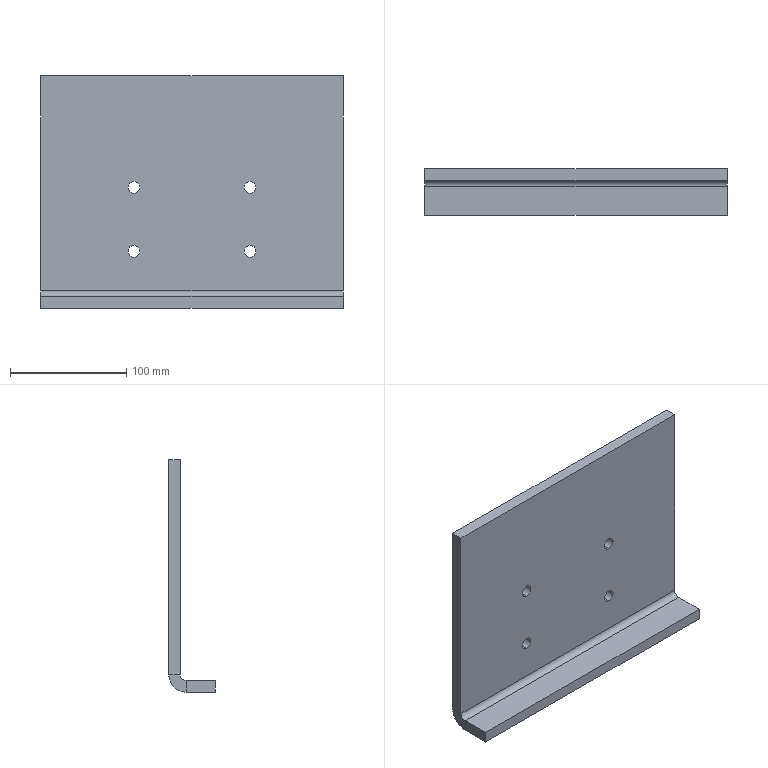Component | SolidWorks | THK-A1017LeftAndRightRectangularTubeConnectingPlate-1 | 1 solid | 22 faces | box 260 x 40 x 200 mm | volume 583572 mm3 | plane 12 | cylinder 10 | commonest cylinder face diameters 10.2 x8 30 x1 10 x1 | material Q235A
STEP:
#1=CARTESIAN_POINT('',(1.969,-2.953,-28.421));
#2=VERTEX_POINT('',#1);
#3=CARTESIAN_POINT('',(1.969,-2.953,-28.823));
#4=VERTEX_POINT('',#3);
#5=CARTESIAN_POINT('',(1.969,-2.953,-28.622));
#6=DIRECTION('',(0.,-1.,0.));
#7=DIRECTION('',(0.,0.,-1.));
#8=AXIS2_PLACEMENT_3D('',#5,#6,#7);
#9=CIRCLE('',#8,0.2008);
#10=EDGE_CURVE('',#2,#4,#9,.T.);
#11=ORIENTED_EDGE('',*,*,#10,.F.);
#12=CARTESIAN_POINT('',(1.969,-3.346,-28.421));
#13=VERTEX_POINT('',#12);
#14=CARTESIAN_POINT('',(1.969,-3.346,-28.421));
#15=DIRECTION('',(0.,-1.,0.));
#16=VECTOR('',#15,39.37);
#17=LINE('',#14,#16);
#18=EDGE_CURVE('',#2,#13,#17,.T.);
#19=ORIENTED_EDGE('',*,*,#18,.T.);
#20=CARTESIAN_POINT('',(1.969,-3.346,-28.823));
#21=VERTEX_POINT('',#20);
#22=CARTESIAN_POINT('',(1.969,-3.346,-28.622));
#23=DIRECTION('',(0.,-1.,0.));
#24=DIRECTION('',(0.,0.,-1.));
#25=AXIS2_PLACEMENT_3D('',#22,#23,#24);
#26=CIRCLE('',#25,0.2008);
#27=EDGE_CURVE('',#13,#21,#26,.T.);
#28=ORIENTED_EDGE('',*,*,#27,.T.);
#29=CARTESIAN_POINT('',(1.969,-3.346,-28.823));
#30=DIRECTION('',(0.,-1.,0.));
#31=VECTOR('',#30,39.37);
#32=LINE('',#29,#31);
#33=EDGE_CURVE('',#4,#21,#32,.T.);
#34=ORIENTED_EDGE('',*,*,#33,.F.);
#35=EDGE_LOOP('',(#11,#19,#28,#34));
#36=FACE_OUTER_BOUND('',#35,.T.);
#37=CARTESIAN_POINT('',(1.969,-3.346,-28.622));
#38=DIRECTION('',(0.,-1.,0.));
#39=DIRECTION('',(0.,0.,-1.));
#40=AXIS2_PLACEMENT_3D('',#37,#38,#39);
#41=CYLINDRICAL_SURFACE('',#40,0.2008);
#42=ADVANCED_FACE('',(#36),#41,.F.);
#43=CARTESIAN_POINT('',(1.969,-2.953,-26.256));
#44=VERTEX_POINT('',#43);
#45=CARTESIAN_POINT('',(1.969,-2.953,-26.657));
#46=VERTEX_POINT('',#45);
#47=CARTESIAN_POINT('',(1.969,-2.953,-26.457));
#48=DIRECTION('',(0.,-1.,0.));
#49=DIRECTION('',(0.,0.,-1.));
#50=AXIS2_PLACEMENT_3D('',#47,#48,#49);
#51=CIRCLE('',#50,0.2008);
#52=EDGE_CURVE('',#44,#46,#51,.T.);
#53=ORIENTED_EDGE('',*,*,#52,.F.);
#54=CARTESIAN_POINT('',(1.969,-3.346,-26.256));
#55=VERTEX_POINT('',#54);
#56=CARTESIAN_POINT('',(1.969,-3.346,-26.256));
#57=DIRECTION('',(0.,-1.,0.));
#58=VECTOR('',#57,39.37);
#59=LINE('',#56,#58);
#60=EDGE_CURVE('',#44,#55,#59,.T.);
#61=ORIENTED_EDGE('',*,*,#60,.T.);
#62=CARTESIAN_POINT('',(1.969,-3.346,-26.657));
#63=VERTEX_POINT('',#62);
#64=CARTESIAN_POINT('',(1.969,-3.346,-26.457));
#65=DIRECTION('',(0.,-1.,0.));
#66=DIRECTION('',(0.,0.,-1.));
#67=AXIS2_PLACEMENT_3D('',#64,#65,#66);
#68=CIRCLE('',#67,0.2008);
#69=EDGE_CURVE('',#55,#63,#68,.T.);
#70=ORIENTED_EDGE('',*,*,#69,.T.);
#71=CARTESIAN_POINT('',(1.969,-3.346,-26.657));
#72=DIRECTION('',(0.,-1.,0.));
#73=VECTOR('',#72,39.37);
#74=LINE('',#71,#73);
#75=EDGE_CURVE('',#46,#63,#74,.T.);
#76=ORIENTED_EDGE('',*,*,#75,.F.);
#77=EDGE_LOOP('',(#53,#61,#70,#76));
#78=FACE_OUTER_BOUND('',#77,.T.);
#79=CARTESIAN_POINT('',(1.969,-3.346,-26.457));
#80=DIRECTION('',(0.,-1.,0.));
#81=DIRECTION('',(0.,0.,-1.));
#82=AXIS2_PLACEMENT_3D('',#79,#80,#81);
#83=CYLINDRICAL_SURFACE('',#82,0.2008);
#84=ADVANCED_FACE('',(#78),#83,.F.);
#85=CARTESIAN_POINT('',(-1.969,-2.953,-26.256));
#86=VERTEX_POINT('',#85);
#87=CARTESIAN_POINT('',(-1.969,-2.953,-26.657));
#88=VERTEX_POINT('',#87);
#89=CARTESIAN_POINT('',(-1.969,-2.953,-26.457));
#90=DIRECTION('',(0.,-1.,0.));
#91=DIRECTION('',(0.,0.,-1.));
#92=AXIS2_PLACEMENT_3D('',#89,#90,#91);
#93=CIRCLE('',#92,0.2008);
#94=EDGE_CURVE('',#86,#88,#93,.T.);
#95=ORIENTED_EDGE('',*,*,#94,.F.);
#96=CARTESIAN_POINT('',(-1.969,-3.346,-26.256));
#97=VERTEX_POINT('',#96);
#98=CARTESIAN_POINT('',(-1.969,-3.346,-26.256));
#99=DIRECTION('',(0.,-1.,0.));
#100=VECTOR('',#99,39.37);
#101=LINE('',#98,#100);
#102=EDGE_CURVE('',#86,#97,#101,.T.);
#103=ORIENTED_EDGE('',*,*,#102,.T.);
#104=CARTESIAN_POINT('',(-1.969,-3.346,-26.657));
#105=VERTEX_POINT('',#104);
#106=CARTESIAN_POINT('',(-1.969,-3.346,-26.457));
#107=DIRECTION('',(0.,-1.,0.));
#108=DIRECTION('',(0.,0.,-1.));
#109=AXIS2_PLACEMENT_3D('',#106,#107,#108);
#110=CIRCLE('',#109,0.2008);
#111=EDGE_CURVE('',#97,#105,#110,.T.);
#112=ORIENTED_EDGE('',*,*,#111,.T.);
#113=CARTESIAN_POINT('',(-1.969,-3.346,-26.657));
#114=DIRECTION('',(0.,-1.,0.));
#115=VECTOR('',#114,39.37);
#116=LINE('',#113,#115);
#117=EDGE_CURVE('',#88,#105,#116,.T.);
#118=ORIENTED_EDGE('',*,*,#117,.F.);
#119=EDGE_LOOP('',(#95,#103,#112,#118));
#120=FACE_OUTER_BOUND('',#119,.T.);
#121=CARTESIAN_POINT('',(-1.969,-3.346,-26.457));
#122=DIRECTION('',(0.,-1.,0.));
#123=DIRECTION('',(0.,0.,-1.));
#124=AXIS2_PLACEMENT_3D('',#121,#122,#123);
#125=CYLINDRICAL_SURFACE('',#124,0.2008);
#126=ADVANCED_FACE('',(#120),#125,.F.);
#127=CARTESIAN_POINT('',(-1.969,-2.953,-28.421));
#128=VERTEX_POINT('',#127);
#129=CARTESIAN_POINT('',(-1.969,-2.953,-28.823));
#130=VERTEX_POINT('',#129);
#131=CARTESIAN_POINT('',(-1.969,-2.953,-28.622));
#132=DIRECTION('',(0.,-1.,0.));
#133=DIRECTION('',(0.,0.,-1.));
#134=AXIS2_PLACEMENT_3D('',#131,#132,#133);
#135=CIRCLE('',#134,0.2008);
#136=EDGE_CURVE('',#128,#130,#135,.T.);
#137=ORIENTED_EDGE('',*,*,#136,.F.);
#138=CARTESIAN_POINT('',(-1.969,-3.346,-28.421));
#139=VERTEX_POINT('',#138);
#140=CARTESIAN_POINT('',(-1.969,-3.346,-28.421));
#141=DIRECTION('',(0.,-1.,0.));
#142=VECTOR('',#141,39.37);
#143=LINE('',#140,#142);
#144=EDGE_CURVE('',#128,#139,#143,.T.);
#145=ORIENTED_EDGE('',*,*,#144,.T.);
#146=CARTESIAN_POINT('',(-1.969,-3.346,-28.823));
#147=VERTEX_POINT('',#146);
#148=CARTESIAN_POINT('',(-1.969,-3.346,-28.622));
#149=DIRECTION('',(0.,-1.,0.));
#150=DIRECTION('',(0.,0.,-1.));
#151=AXIS2_PLACEMENT_3D('',#148,#149,#150);
#152=CIRCLE('',#151,0.2008);
#153=EDGE_CURVE('',#139,#147,#152,.T.);
#154=ORIENTED_EDGE('',*,*,#153,.T.);
#155=CARTESIAN_POINT('',(-1.969,-3.346,-28.823));
#156=DIRECTION('',(0.,-1.,0.));
#157=VECTOR('',#156,39.37);
#158=LINE('',#155,#157);
#159=EDGE_CURVE('',#130,#147,#158,.T.);
#160=ORIENTED_EDGE('',*,*,#159,.F.);
#161=EDGE_LOOP('',(#137,#145,#154,#160));
#162=FACE_OUTER_BOUND('',#161,.T.);
#163=CARTESIAN_POINT('',(-1.969,-3.346,-28.622));
#164=DIRECTION('',(0.,-1.,0.));
#165=DIRECTION('',(0.,0.,-1.));
#166=AXIS2_PLACEMENT_3D('',#163,#164,#165);
#167=CYLINDRICAL_SURFACE('',#166,0.2008);
#168=ADVANCED_FACE('',(#162),#167,.F.);
#169=CARTESIAN_POINT('',(5.118,-3.543,-30.551));
#170=VERTEX_POINT('',#169);
#171=CARTESIAN_POINT('',(5.118,-3.543,-30.157));
#172=VERTEX_POINT('',#171);
#173=CARTESIAN_POINT('',(5.118,-3.543,-30.551));
#174=DIRECTION('',(0.,-0.,1.));
#175=VECTOR('',#174,39.37);
#176=LINE('',#173,#175);
#177=EDGE_CURVE('',#170,#172,#176,.T.);
#178=ORIENTED_EDGE('',*,*,#177,.F.);
#179=CARTESIAN_POINT('',(5.118,-2.953,-29.961));
#180=VERTEX_POINT('',#179);
#181=CARTESIAN_POINT('',(5.118,-3.543,-29.961));
#182=DIRECTION('',(-1.,0.,0.));
#183=DIRECTION('',(0.,0.,-1.));
#184=AXIS2_PLACEMENT_3D('',#181,#182,#183);
#185=CIRCLE('',#184,0.5906);
#186=EDGE_CURVE('',#180,#170,#185,.T.);
#187=ORIENTED_EDGE('',*,*,#186,.F.);
#188=CARTESIAN_POINT('',(5.118,-3.346,-29.961));
#189=VERTEX_POINT('',#188);
#190=CARTESIAN_POINT('',(5.118,-3.346,-29.961));
#191=DIRECTION('',(0.,1.,-0.));
#192=VECTOR('',#191,39.37);
#193=LINE('',#190,#192);
#194=EDGE_CURVE('',#189,#180,#193,.T.);
#195=ORIENTED_EDGE('',*,*,#194,.F.);
#196=CARTESIAN_POINT('',(5.118,-3.543,-29.961));
#197=DIRECTION('',(-1.,0.,0.));
#198=DIRECTION('',(0.,0.,-1.));
#199=AXIS2_PLACEMENT_3D('',#196,#197,#198);
#200=CIRCLE('',#199,0.1969);
#201=EDGE_CURVE('',#189,#172,#200,.T.);
#202=ORIENTED_EDGE('',*,*,#201,.T.);
#203=EDGE_LOOP('',(#178,#187,#195,#202));
#204=FACE_OUTER_BOUND('',#203,.T.);
#205=CARTESIAN_POINT('',(5.118,-3.543,-30.551));
#206=DIRECTION('',(1.,0.,0.));
#207=DIRECTION('',(0.,0.,-1.));
#208=AXIS2_PLACEMENT_3D('',#205,#206,#207);
#209=PLANE('',#208);
#210=ADVANCED_FACE('',(#204),#209,.T.);
#211=CARTESIAN_POINT('',(5.118,-4.528,-30.551));
#212=VERTEX_POINT('',#211);
#213=CARTESIAN_POINT('',(5.118,-2.953,-30.551));
#214=DIRECTION('',(0.,-1.,-0.));
#215=VECTOR('',#214,39.37);
#216=LINE('',#213,#215);
#217=EDGE_CURVE('',#170,#212,#216,.T.);
#218=ORIENTED_EDGE('',*,*,#217,.F.);
#219=ORIENTED_EDGE('',*,*,#177,.T.);
#220=CARTESIAN_POINT('',(5.118,-4.528,-30.157));
#221=VERTEX_POINT('',#220);
#222=CARTESIAN_POINT('',(5.118,-2.953,-30.157));
#223=DIRECTION('',(0.,-1.,-0.));
#224=VECTOR('',#223,39.37);
#225=LINE('',#222,#224);
#226=EDGE_CURVE('',#172,#221,#225,.T.);
#227=ORIENTED_EDGE('',*,*,#226,.T.);
#228=CARTESIAN_POINT('',(5.118,-4.528,-30.551));
#229=DIRECTION('',(0.,0.,1.));
#230=VECTOR('',#229,39.37);
#231=LINE('',#228,#230);
#232=EDGE_CURVE('',#212,#221,#231,.T.);
#233=ORIENTED_EDGE('',*,*,#232,.F.);
#234=EDGE_LOOP('',(#218,#219,#227,#233));
#235=FACE_OUTER_BOUND('',#234,.T.);
#236=CARTESIAN_POINT('',(5.118,-3.346,-29.961));
#237=DIRECTION('',(1.,0.,0.));
#238=DIRECTION('',(0.,0.,-1.));
#239=AXIS2_PLACEMENT_3D('',#236,#237,#238);
#240=PLANE('',#239);
#241=ADVANCED_FACE('',(#235),#240,.T.);
#242=CARTESIAN_POINT('',(-5.118,-2.953,-29.961));
#243=VERTEX_POINT('',#242);
#244=CARTESIAN_POINT('',(-5.118,-3.346,-29.961));
#245=VERTEX_POINT('',#244);
#246=CARTESIAN_POINT('',(-5.118,-2.953,-29.961));
#247=DIRECTION('',(0.,-1.,0.));
#248=VECTOR('',#247,39.37);
#249=LINE('',#246,#248);
#250=EDGE_CURVE('',#243,#245,#249,.T.);
#251=ORIENTED_EDGE('',*,*,#250,.F.);
#252=CARTESIAN_POINT('',(-5.118,-3.543,-30.551));
#253=VERTEX_POINT('',#252);
#254=CARTESIAN_POINT('',(-5.118,-3.543,-29.961));
#255=DIRECTION('',(-1.,0.,0.));
#256=DIRECTION('',(0.,0.,-1.));
#257=AXIS2_PLACEMENT_3D('',#254,#255,#256);
#258=CIRCLE('',#257,0.5906);
#259=EDGE_CURVE('',#243,#253,#258,.T.);
#260=ORIENTED_EDGE('',*,*,#259,.T.);
#261=CARTESIAN_POINT('',(-5.118,-3.543,-30.157));
#262=VERTEX_POINT('',#261);
#263=CARTESIAN_POINT('',(-5.118,-3.543,-30.157));
#264=DIRECTION('',(0.,0.,-1.));
#265=VECTOR('',#264,39.37);
#266=LINE('',#263,#265);
#267=EDGE_CURVE('',#262,#253,#266,.T.);
#268=ORIENTED_EDGE('',*,*,#267,.F.);
#269=CARTESIAN_POINT('',(-5.118,-3.543,-29.961));
#270=DIRECTION('',(-1.,0.,0.));
#271=DIRECTION('',(0.,0.,-1.));
#272=AXIS2_PLACEMENT_3D('',#269,#270,#271);
#273=CIRCLE('',#272,0.1969);
#274=EDGE_CURVE('',#245,#262,#273,.T.);
#275=ORIENTED_EDGE('',*,*,#274,.F.);
#276=EDGE_LOOP('',(#251,#260,#268,#275));
#277=FACE_OUTER_BOUND('',#276,.T.);
#278=CARTESIAN_POINT('',(-5.118,-2.953,-29.961));
#279=DIRECTION('',(-1.,0.,0.));
#280=DIRECTION('',(0.,0.,1.));
#281=AXIS2_PLACEMENT_3D('',#278,#279,#280);
#282=PLANE('',#281);
#283=ADVANCED_FACE('',(#277),#282,.T.);
#284=CARTESIAN_POINT('',(-5.118,-2.953,-22.677));
#285=VERTEX_POINT('',#284);
#286=CARTESIAN_POINT('',(-5.118,-2.953,-22.677));
#287=DIRECTION('',(0.,0.,-1.));
#288=VECTOR('',#287,39.37);
#289=LINE('',#286,#288);
#290=EDGE_CURVE('',#285,#243,#289,.T.);
#291=ORIENTED_EDGE('',*,*,#290,.T.);
#292=ORIENTED_EDGE('',*,*,#250,.T.);
#293=CARTESIAN_POINT('',(-5.118,-3.346,-22.677));
#294=VERTEX_POINT('',#293);
#295=CARTESIAN_POINT('',(-5.118,-3.346,-22.677));
#296=DIRECTION('',(0.,0.,-1.));
#297=VECTOR('',#296,39.37);
#298=LINE('',#295,#297);
#299=EDGE_CURVE('',#294,#245,#298,.T.);
#300=ORIENTED_EDGE('',*,*,#299,.F.);
#301=CARTESIAN_POINT('',(-5.118,-3.346,-22.677));
#302=DIRECTION('',(0.,1.,0.));
#303=VECTOR('',#302,39.37);
#304=LINE('',#301,#303);
#305=EDGE_CURVE('',#294,#285,#304,.T.);
#306=ORIENTED_EDGE('',*,*,#305,.T.);
#307=EDGE_LOOP('',(#291,#292,#300,#306));
#308=FACE_OUTER_BOUND('',#307,.T.);
#309=CARTESIAN_POINT('',(-5.118,-3.543,-30.157));
#310=DIRECTION('',(-1.,0.,0.));
#311=DIRECTION('',(0.,0.,1.));
#312=AXIS2_PLACEMENT_3D('',#309,#310,#311);
#313=PLANE('',#312);
#314=ADVANCED_FACE('',(#308),#313,.T.);
#315=CARTESIAN_POINT('',(-5.118,-4.528,-30.157));
#316=VERTEX_POINT('',#315);
#317=CARTESIAN_POINT('',(-5.118,-2.953,-30.157));
#318=DIRECTION('',(0.,-1.,-0.));
#319=VECTOR('',#318,39.37);
#320=LINE('',#317,#319);
#321=EDGE_CURVE('',#262,#316,#320,.T.);
#322=ORIENTED_EDGE('',*,*,#321,.T.);
#323=CARTESIAN_POINT('',(5.118,-4.528,-30.157));
#324=DIRECTION('',(-1.,0.,0.));
#325=VECTOR('',#324,39.37);
#326=LINE('',#323,#325);
#327=EDGE_CURVE('',#221,#316,#326,.T.);
#328=ORIENTED_EDGE('',*,*,#327,.F.);
#329=ORIENTED_EDGE('',*,*,#226,.F.);
#330=CARTESIAN_POINT('',(5.118,-3.543,-30.157));
#331=DIRECTION('',(-1.,0.,0.));
#332=VECTOR('',#331,39.37);
#333=LINE('',#330,#332);
#334=EDGE_CURVE('',#172,#262,#333,.T.);
#335=ORIENTED_EDGE('',*,*,#334,.T.);
#336=EDGE_LOOP('',(#322,#328,#329,#335));
#337=FACE_OUTER_BOUND('',#336,.T.);
#338=CARTESIAN_POINT('',(5.118,-2.953,-30.157));
#339=DIRECTION('',(0.,0.,-1.));
#340=DIRECTION('',(0.,1.,0.));
#341=AXIS2_PLACEMENT_3D('',#338,#339,#340);
#342=PLANE('',#341);
#343=ADVANCED_FACE('',(#337),#342,.F.);
#344=CARTESIAN_POINT('',(-5.118,-4.528,-30.551));
#345=VERTEX_POINT('',#344);
#346=CARTESIAN_POINT('',(-5.118,-4.528,-30.551));
#347=DIRECTION('',(0.,0.,1.));
#348=VECTOR('',#347,39.37);
#349=LINE('',#346,#348);
#350=EDGE_CURVE('',#345,#316,#349,.T.);
#351=ORIENTED_EDGE('',*,*,#350,.F.);
#352=CARTESIAN_POINT('',(5.118,-4.528,-30.551));
#353=DIRECTION('',(-1.,0.,0.));
#354=VECTOR('',#353,39.37);
#355=LINE('',#352,#354);
#356=EDGE_CURVE('',#212,#345,#355,.T.);
#357=ORIENTED_EDGE('',*,*,#356,.F.);
#358=ORIENTED_EDGE('',*,*,#232,.T.);
#359=ORIENTED_EDGE('',*,*,#327,.T.);
#360=EDGE_LOOP('',(#351,#357,#358,#359));
#361=FACE_OUTER_BOUND('',#360,.T.);
#362=CARTESIAN_POINT('',(5.118,-4.528,-30.551));
#363=DIRECTION('',(0.,-1.,0.));
#364=DIRECTION('',(0.,0.,-1.));
#365=AXIS2_PLACEMENT_3D('',#362,#363,#364);
#366=PLANE('',#365);
#367=ADVANCED_FACE('',(#361),#366,.T.);
#368=CARTESIAN_POINT('',(-5.118,-2.953,-30.551));
#369=DIRECTION('',(0.,-1.,-0.));
#370=VECTOR('',#369,39.37);
#371=LINE('',#368,#370);
#372=EDGE_CURVE('',#253,#345,#371,.T.);
#373=ORIENTED_EDGE('',*,*,#372,.F.);
#374=CARTESIAN_POINT('',(5.118,-3.543,-30.551));
#375=DIRECTION('',(-1.,0.,0.));
#376=VECTOR('',#375,39.37);
#377=LINE('',#374,#376);
#378=EDGE_CURVE('',#170,#253,#377,.T.);
#379=ORIENTED_EDGE('',*,*,#378,.F.);
#380=ORIENTED_EDGE('',*,*,#217,.T.);
#381=ORIENTED_EDGE('',*,*,#356,.T.);
#382=EDGE_LOOP('',(#373,#379,#380,#381));
#383=FACE_OUTER_BOUND('',#382,.T.);
#384=CARTESIAN_POINT('',(5.118,-2.953,-30.551));
#385=DIRECTION('',(0.,0.,-1.));
#386=DIRECTION('',(0.,1.,0.));
#387=AXIS2_PLACEMENT_3D('',#384,#385,#386);
#388=PLANE('',#387);
#389=ADVANCED_FACE('',(#383),#388,.T.);
#390=ORIENTED_EDGE('',*,*,#259,.F.);
#391=CARTESIAN_POINT('',(5.118,-2.953,-29.961));
#392=DIRECTION('',(-1.,0.,0.));
#393=VECTOR('',#392,39.37);
#394=LINE('',#391,#393);
#395=EDGE_CURVE('',#180,#243,#394,.T.);
#396=ORIENTED_EDGE('',*,*,#395,.F.);
#397=ORIENTED_EDGE('',*,*,#186,.T.);
#398=ORIENTED_EDGE('',*,*,#378,.T.);
#399=EDGE_LOOP('',(#390,#396,#397,#398));
#400=FACE_OUTER_BOUND('',#399,.T.);
#401=CARTESIAN_POINT('',(5.118,-3.543,-29.961));
#402=DIRECTION('',(-1.,0.,0.));
#403=DIRECTION('',(0.,0.,1.));
#404=AXIS2_PLACEMENT_3D('',#401,#402,#403);
#405=CYLINDRICAL_SURFACE('',#404,0.5906);
#406=ADVANCED_FACE('',(#400),#405,.T.);
#407=CARTESIAN_POINT('',(1.969,-2.953,-28.622));
#408=DIRECTION('',(0.,-1.,0.));
#409=DIRECTION('',(0.,0.,-1.));
#410=AXIS2_PLACEMENT_3D('',#407,#408,#409);
#411=CIRCLE('',#410,0.2008);
#412=EDGE_CURVE('',#4,#2,#411,.T.);
#413=ORIENTED_EDGE('',*,*,#412,.T.);
#414=ORIENTED_EDGE('',*,*,#10,.T.);
#415=EDGE_LOOP('',(#413,#414));
#416=FACE_BOUND('',#415,.T.);
#417=CARTESIAN_POINT('',(1.969,-2.953,-26.457));
#418=DIRECTION('',(0.,-1.,0.));
#419=DIRECTION('',(0.,0.,-1.));
#420=AXIS2_PLACEMENT_3D('',#417,#418,#419);
#421=CIRCLE('',#420,0.2008);
#422=EDGE_CURVE('',#46,#44,#421,.T.);
#423=ORIENTED_EDGE('',*,*,#422,.T.);
#424=ORIENTED_EDGE('',*,*,#52,.T.);
#425=EDGE_LOOP('',(#423,#424));
#426=FACE_BOUND('',#425,.T.);
#427=CARTESIAN_POINT('',(-1.969,-2.953,-26.457));
#428=DIRECTION('',(0.,-1.,0.));
#429=DIRECTION('',(0.,0.,-1.));
#430=AXIS2_PLACEMENT_3D('',#427,#428,#429);
#431=CIRCLE('',#430,0.2008);
#432=EDGE_CURVE('',#88,#86,#431,.T.);
#433=ORIENTED_EDGE('',*,*,#432,.T.);
#434=ORIENTED_EDGE('',*,*,#94,.T.);
#435=EDGE_LOOP('',(#433,#434));
#436=FACE_BOUND('',#435,.T.);
#437=CARTESIAN_POINT('',(-1.969,-2.953,-28.622));
#438=DIRECTION('',(0.,-1.,0.));
#439=DIRECTION('',(0.,0.,-1.));
#440=AXIS2_PLACEMENT_3D('',#437,#438,#439);
#441=CIRCLE('',#440,0.2008);
#442=EDGE_CURVE('',#130,#128,#441,.T.);
#443=ORIENTED_EDGE('',*,*,#442,.T.);
#444=ORIENTED_EDGE('',*,*,#136,.T.);
#445=EDGE_LOOP('',(#443,#444));
#446=FACE_BOUND('',#445,.T.);
#447=ORIENTED_EDGE('',*,*,#290,.F.);
#448=CARTESIAN_POINT('',(5.118,-2.953,-22.677));
#449=VERTEX_POINT('',#448);
#450=CARTESIAN_POINT('',(5.118,-2.953,-22.677));
#451=DIRECTION('',(-1.,0.,0.));
#452=VECTOR('',#451,39.37);
#453=LINE('',#450,#452);
#454=EDGE_CURVE('',#449,#285,#453,.T.);
#455=ORIENTED_EDGE('',*,*,#454,.F.);
#456=CARTESIAN_POINT('',(5.118,-2.953,-22.677));
#457=DIRECTION('',(0.,0.,-1.));
#458=VECTOR('',#457,39.37);
#459=LINE('',#456,#458);
#460=EDGE_CURVE('',#449,#180,#459,.T.);
#461=ORIENTED_EDGE('',*,*,#460,.T.);
#462=ORIENTED_EDGE('',*,*,#395,.T.);
#463=EDGE_LOOP('',(#447,#455,#461,#462));
#464=FACE_OUTER_BOUND('',#463,.T.);
#465=CARTESIAN_POINT('',(5.118,-2.953,-22.677));
#466=DIRECTION('',(0.,1.,0.));
#467=DIRECTION('',(0.,0.,1.));
#468=AXIS2_PLACEMENT_3D('',#465,#466,#467);
#469=PLANE('',#468);
#470=ADVANCED_FACE('',(#416,#426,#436,#446,#464),#469,.T.);
#471=ORIENTED_EDGE('',*,*,#305,.F.);
#472=CARTESIAN_POINT('',(5.118,-3.346,-22.677));
#473=VERTEX_POINT('',#472);
#474=CARTESIAN_POINT('',(5.118,-3.346,-22.677));
#475=DIRECTION('',(-1.,0.,0.));
#476=VECTOR('',#475,39.37);
#477=LINE('',#474,#476);
#478=EDGE_CURVE('',#473,#294,#477,.T.);
#479=ORIENTED_EDGE('',*,*,#478,.F.);
#480=CARTESIAN_POINT('',(5.118,-3.346,-22.677));
#481=DIRECTION('',(0.,1.,0.));
#482=VECTOR('',#481,39.37);
#483=LINE('',#480,#482);
#484=EDGE_CURVE('',#473,#449,#483,.T.);
#485=ORIENTED_EDGE('',*,*,#484,.T.);
#486=ORIENTED_EDGE('',*,*,#454,.T.);
#487=EDGE_LOOP('',(#471,#479,#485,#486));
#488=FACE_OUTER_BOUND('',#487,.T.);
#489=CARTESIAN_POINT('',(5.118,-3.346,-22.677));
#490=DIRECTION('',(0.,0.,1.));
#491=DIRECTION('',(1.,0.,0.));
#492=AXIS2_PLACEMENT_3D('',#489,#490,#491);
#493=PLANE('',#492);
#494=ADVANCED_FACE('',(#488),#493,.T.);
#495=CARTESIAN_POINT('',(1.969,-3.346,-28.622));
#496=DIRECTION('',(0.,-1.,0.));
#497=DIRECTION('',(0.,0.,-1.));
#498=AXIS2_PLACEMENT_3D('',#495,#496,#497);
#499=CIRCLE('',#498,0.2008);
#500=EDGE_CURVE('',#21,#13,#499,.T.);
#501=ORIENTED_EDGE('',*,*,#500,.F.);
#502=ORIENTED_EDGE('',*,*,#27,.F.);
#503=EDGE_LOOP('',(#501,#502));
#504=FACE_BOUND('',#503,.T.);
#505=CARTESIAN_POINT('',(1.969,-3.346,-26.457));
#506=DIRECTION('',(0.,-1.,0.));
#507=DIRECTION('',(0.,0.,-1.));
#508=AXIS2_PLACEMENT_3D('',#505,#506,#507);
#509=CIRCLE('',#508,0.2008);
#510=EDGE_CURVE('',#63,#55,#509,.T.);
#511=ORIENTED_EDGE('',*,*,#510,.F.);
#512=ORIENTED_EDGE('',*,*,#69,.F.);
#513=EDGE_LOOP('',(#511,#512));
#514=FACE_BOUND('',#513,.T.);
#515=CARTESIAN_POINT('',(-1.969,-3.346,-26.457));
#516=DIRECTION('',(0.,-1.,0.));
#517=DIRECTION('',(0.,0.,-1.));
#518=AXIS2_PLACEMENT_3D('',#515,#516,#517);
#519=CIRCLE('',#518,0.2008);
#520=EDGE_CURVE('',#105,#97,#519,.T.);
#521=ORIENTED_EDGE('',*,*,#520,.F.);
#522=ORIENTED_EDGE('',*,*,#111,.F.);
#523=EDGE_LOOP('',(#521,#522));
#524=FACE_BOUND('',#523,.T.);
#525=CARTESIAN_POINT('',(-1.969,-3.346,-28.622));
#526=DIRECTION('',(0.,-1.,0.));
#527=DIRECTION('',(0.,0.,-1.));
#528=AXIS2_PLACEMENT_3D('',#525,#526,#527);
#529=CIRCLE('',#528,0.2008);
#530=EDGE_CURVE('',#147,#139,#529,.T.);
#531=ORIENTED_EDGE('',*,*,#530,.F.);
#532=ORIENTED_EDGE('',*,*,#153,.F.);
#533=EDGE_LOOP('',(#531,#532));
#534=FACE_BOUND('',#533,.T.);
#535=ORIENTED_EDGE('',*,*,#299,.T.);
#536=CARTESIAN_POINT('',(5.118,-3.346,-29.961));
#537=DIRECTION('',(-1.,0.,0.));
#538=VECTOR('',#537,39.37);
#539=LINE('',#536,#538);
#540=EDGE_CURVE('',#189,#245,#539,.T.);
#541=ORIENTED_EDGE('',*,*,#540,.F.);
#542=CARTESIAN_POINT('',(5.118,-3.346,-22.677));
#543=DIRECTION('',(0.,0.,-1.));
#544=VECTOR('',#543,39.37);
#545=LINE('',#542,#544);
#546=EDGE_CURVE('',#473,#189,#545,.T.);
#547=ORIENTED_EDGE('',*,*,#546,.F.);
#548=ORIENTED_EDGE('',*,*,#478,.T.);
#549=EDGE_LOOP('',(#535,#541,#547,#548));
#550=FACE_OUTER_BOUND('',#549,.T.);
#551=CARTESIAN_POINT('',(5.118,-3.346,-22.677));
#552=DIRECTION('',(0.,1.,0.));
#553=DIRECTION('',(0.,0.,1.));
#554=AXIS2_PLACEMENT_3D('',#551,#552,#553);
#555=PLANE('',#554);
#556=ADVANCED_FACE('',(#504,#514,#524,#534,#550),#555,.F.);
#557=ORIENTED_EDGE('',*,*,#274,.T.);
#558=ORIENTED_EDGE('',*,*,#334,.F.);
#559=ORIENTED_EDGE('',*,*,#201,.F.);
#560=ORIENTED_EDGE('',*,*,#540,.T.);
#561=EDGE_LOOP('',(#557,#558,#559,#560));
#562=FACE_OUTER_BOUND('',#561,.T.);
#563=CARTESIAN_POINT('',(5.118,-3.543,-29.961));
#564=DIRECTION('',(-1.,0.,0.));
#565=DIRECTION('',(0.,0.,1.));
#566=AXIS2_PLACEMENT_3D('',#563,#564,#565);
#567=CYLINDRICAL_SURFACE('',#566,0.1969);
#568=ADVANCED_FACE('',(#562),#567,.F.);
#569=ORIENTED_EDGE('',*,*,#546,.T.);
#570=ORIENTED_EDGE('',*,*,#194,.T.);
#571=ORIENTED_EDGE('',*,*,#460,.F.);
#572=ORIENTED_EDGE('',*,*,#484,.F.);
#573=EDGE_LOOP('',(#569,#570,#571,#572));
#574=FACE_OUTER_BOUND('',#573,.T.);
#575=CARTESIAN_POINT('',(5.118,-3.543,-29.961));
#576=DIRECTION('',(1.,0.,0.));
#577=DIRECTION('',(0.,0.,-1.));
#578=AXIS2_PLACEMENT_3D('',#575,#576,#577);
#579=PLANE('',#578);
#580=ADVANCED_FACE('',(#574),#579,.T.);
#581=ORIENTED_EDGE('',*,*,#321,.F.);
#582=ORIENTED_EDGE('',*,*,#267,.T.);
#583=ORIENTED_EDGE('',*,*,#372,.T.);
#584=ORIENTED_EDGE('',*,*,#350,.T.);
#585=EDGE_LOOP('',(#581,#582,#583,#584));
#586=FACE_OUTER_BOUND('',#585,.T.);
#587=CARTESIAN_POINT('',(-5.118,-3.543,-29.961));
#588=DIRECTION('',(1.,0.,0.));
#589=DIRECTION('',(0.,0.,-1.));
#590=AXIS2_PLACEMENT_3D('',#587,#588,#589);
#591=PLANE('',#590);
#592=ADVANCED_FACE('',(#586),#591,.F.);
#593=ORIENTED_EDGE('',*,*,#144,.F.);
#594=ORIENTED_EDGE('',*,*,#442,.F.);
#595=ORIENTED_EDGE('',*,*,#159,.T.);
#596=ORIENTED_EDGE('',*,*,#530,.T.);
#597=EDGE_LOOP('',(#593,#594,#595,#596));
#598=FACE_OUTER_BOUND('',#597,.T.);
#599=CARTESIAN_POINT('',(-1.969,-3.346,-28.622));
#600=DIRECTION('',(0.,-1.,0.));
#601=DIRECTION('',(0.,0.,-1.));
#602=AXIS2_PLACEMENT_3D('',#599,#600,#601);
#603=CYLINDRICAL_SURFACE('',#602,0.2008);
#604=ADVANCED_FACE('',(#598),#603,.F.);
#605=ORIENTED_EDGE('',*,*,#102,.F.);
#606=ORIENTED_EDGE('',*,*,#432,.F.);
#607=ORIENTED_EDGE('',*,*,#117,.T.);
#608=ORIENTED_EDGE('',*,*,#520,.T.);
#609=EDGE_LOOP('',(#605,#606,#607,#608));
#610=FACE_OUTER_BOUND('',#609,.T.);
#611=CARTESIAN_POINT('',(-1.969,-3.346,-26.457));
#612=DIRECTION('',(0.,-1.,0.));
#613=DIRECTION('',(0.,0.,-1.));
#614=AXIS2_PLACEMENT_3D('',#611,#612,#613);
#615=CYLINDRICAL_SURFACE('',#614,0.2008);
#616=ADVANCED_FACE('',(#610),#615,.F.);
#617=ORIENTED_EDGE('',*,*,#60,.F.);
#618=ORIENTED_EDGE('',*,*,#422,.F.);
#619=ORIENTED_EDGE('',*,*,#75,.T.);
#620=ORIENTED_EDGE('',*,*,#510,.T.);
#621=EDGE_LOOP('',(#617,#618,#619,#620));
#622=FACE_OUTER_BOUND('',#621,.T.);
#623=CARTESIAN_POINT('',(1.969,-3.346,-26.457));
#624=DIRECTION('',(0.,-1.,0.));
#625=DIRECTION('',(0.,0.,-1.));
#626=AXIS2_PLACEMENT_3D('',#623,#624,#625);
#627=CYLINDRICAL_SURFACE('',#626,0.2008);
#628=ADVANCED_FACE('',(#622),#627,.F.);
#629=ORIENTED_EDGE('',*,*,#18,.F.);
#630=ORIENTED_EDGE('',*,*,#412,.F.);
#631=ORIENTED_EDGE('',*,*,#33,.T.);
#632=ORIENTED_EDGE('',*,*,#500,.T.);
#633=EDGE_LOOP('',(#629,#630,#631,#632));
#634=FACE_OUTER_BOUND('',#633,.T.);
#635=CARTESIAN_POINT('',(1.969,-3.346,-28.622));
#636=DIRECTION('',(0.,-1.,0.));
#637=DIRECTION('',(0.,0.,-1.));
#638=AXIS2_PLACEMENT_3D('',#635,#636,#637);
#639=CYLINDRICAL_SURFACE('',#638,0.2008);
#640=ADVANCED_FACE('',(#634),#639,.F.);
#641=CLOSED_SHELL('',(#42,#84,#126,#168,#210,#241,#283,#314,#343,#367,#389,#406,#470,#494,#556,#568,#580,#592,#604,#616,#628,#640));
#642=MANIFOLD_SOLID_BREP('',#641);
#643=CARTESIAN_POINT('',(0.,0.,0.));
#644=DIRECTION('',(0.,0.,1.));
#645=DIRECTION('',(1.,0.,0.));
#646=AXIS2_PLACEMENT_3D('',#643,#644,#645);
#647=(LENGTH_UNIT()NAMED_UNIT(*)SI_UNIT($,.METRE.));
#648=LENGTH_MEASURE_WITH_UNIT(LENGTH_MEASURE(0.0254),#647);
#649=DIMENSIONAL_EXPONENTS(1.,0.,0.,0.,0.,0.,0.);
#650=(CONVERSION_BASED_UNIT('',#648)LENGTH_UNIT()NAMED_UNIT(#649));
#651=UNCERTAINTY_MEASURE_WITH_UNIT(LENGTH_MEASURE(0.00001),#650,'','');
#652=(NAMED_UNIT(*)PLANE_ANGLE_UNIT()SI_UNIT($,.RADIAN.));
#653=(NAMED_UNIT(*)SI_UNIT($,.STERADIAN.)SOLID_ANGLE_UNIT());
#654=(GEOMETRIC_REPRESENTATION_CONTEXT(3)GLOBAL_UNCERTAINTY_ASSIGNED_CONTEXT((#651))GLOBAL_UNIT_ASSIGNED_CONTEXT((#650,#652,#653))REPRESENTATION_CONTEXT('',''));
#655=ADVANCED_BREP_SHAPE_REPRESENTATION('',(#642,#646),#654);
#656=COLOUR_RGB('',0.7922,0.8196,0.9333);
#657=FILL_AREA_STYLE_COLOUR('',#656);
#658=FILL_AREA_STYLE('',(#657));
#659=SURFACE_STYLE_FILL_AREA(#658);
#660=SURFACE_SIDE_STYLE('',(#659));
#661=SURFACE_STYLE_USAGE(.BOTH.,#660);
#662=PRESENTATION_STYLE_ASSIGNMENT((#661));
#663=STYLED_ITEM('',(#662),#642);
#664=(LENGTH_UNIT()NAMED_UNIT(*)SI_UNIT($,.METRE.));
#665=LENGTH_MEASURE_WITH_UNIT(LENGTH_MEASURE(0.0254),#664);
#666=DIMENSIONAL_EXPONENTS(1.,0.,0.,0.,0.,0.,0.);
#667=(CONVERSION_BASED_UNIT('',#665)LENGTH_UNIT()NAMED_UNIT(#666));
#668=UNCERTAINTY_MEASURE_WITH_UNIT(LENGTH_MEASURE(0.00001),#667,'','');
#669=(NAMED_UNIT(*)PLANE_ANGLE_UNIT()SI_UNIT($,.RADIAN.));
#670=(NAMED_UNIT(*)SI_UNIT($,.STERADIAN.)SOLID_ANGLE_UNIT());
#671=(GEOMETRIC_REPRESENTATION_CONTEXT(3)GLOBAL_UNCERTAINTY_ASSIGNED_CONTEXT((#668))GLOBAL_UNIT_ASSIGNED_CONTEXT((#667,#669,#670))REPRESENTATION_CONTEXT('',''));
#672=MECHANICAL_DESIGN_GEOMETRIC_PRESENTATION_REPRESENTATION('',(#663),#671);
#673=PRESENTATION_LAYER_ASSIGNMENT('','',(#663));